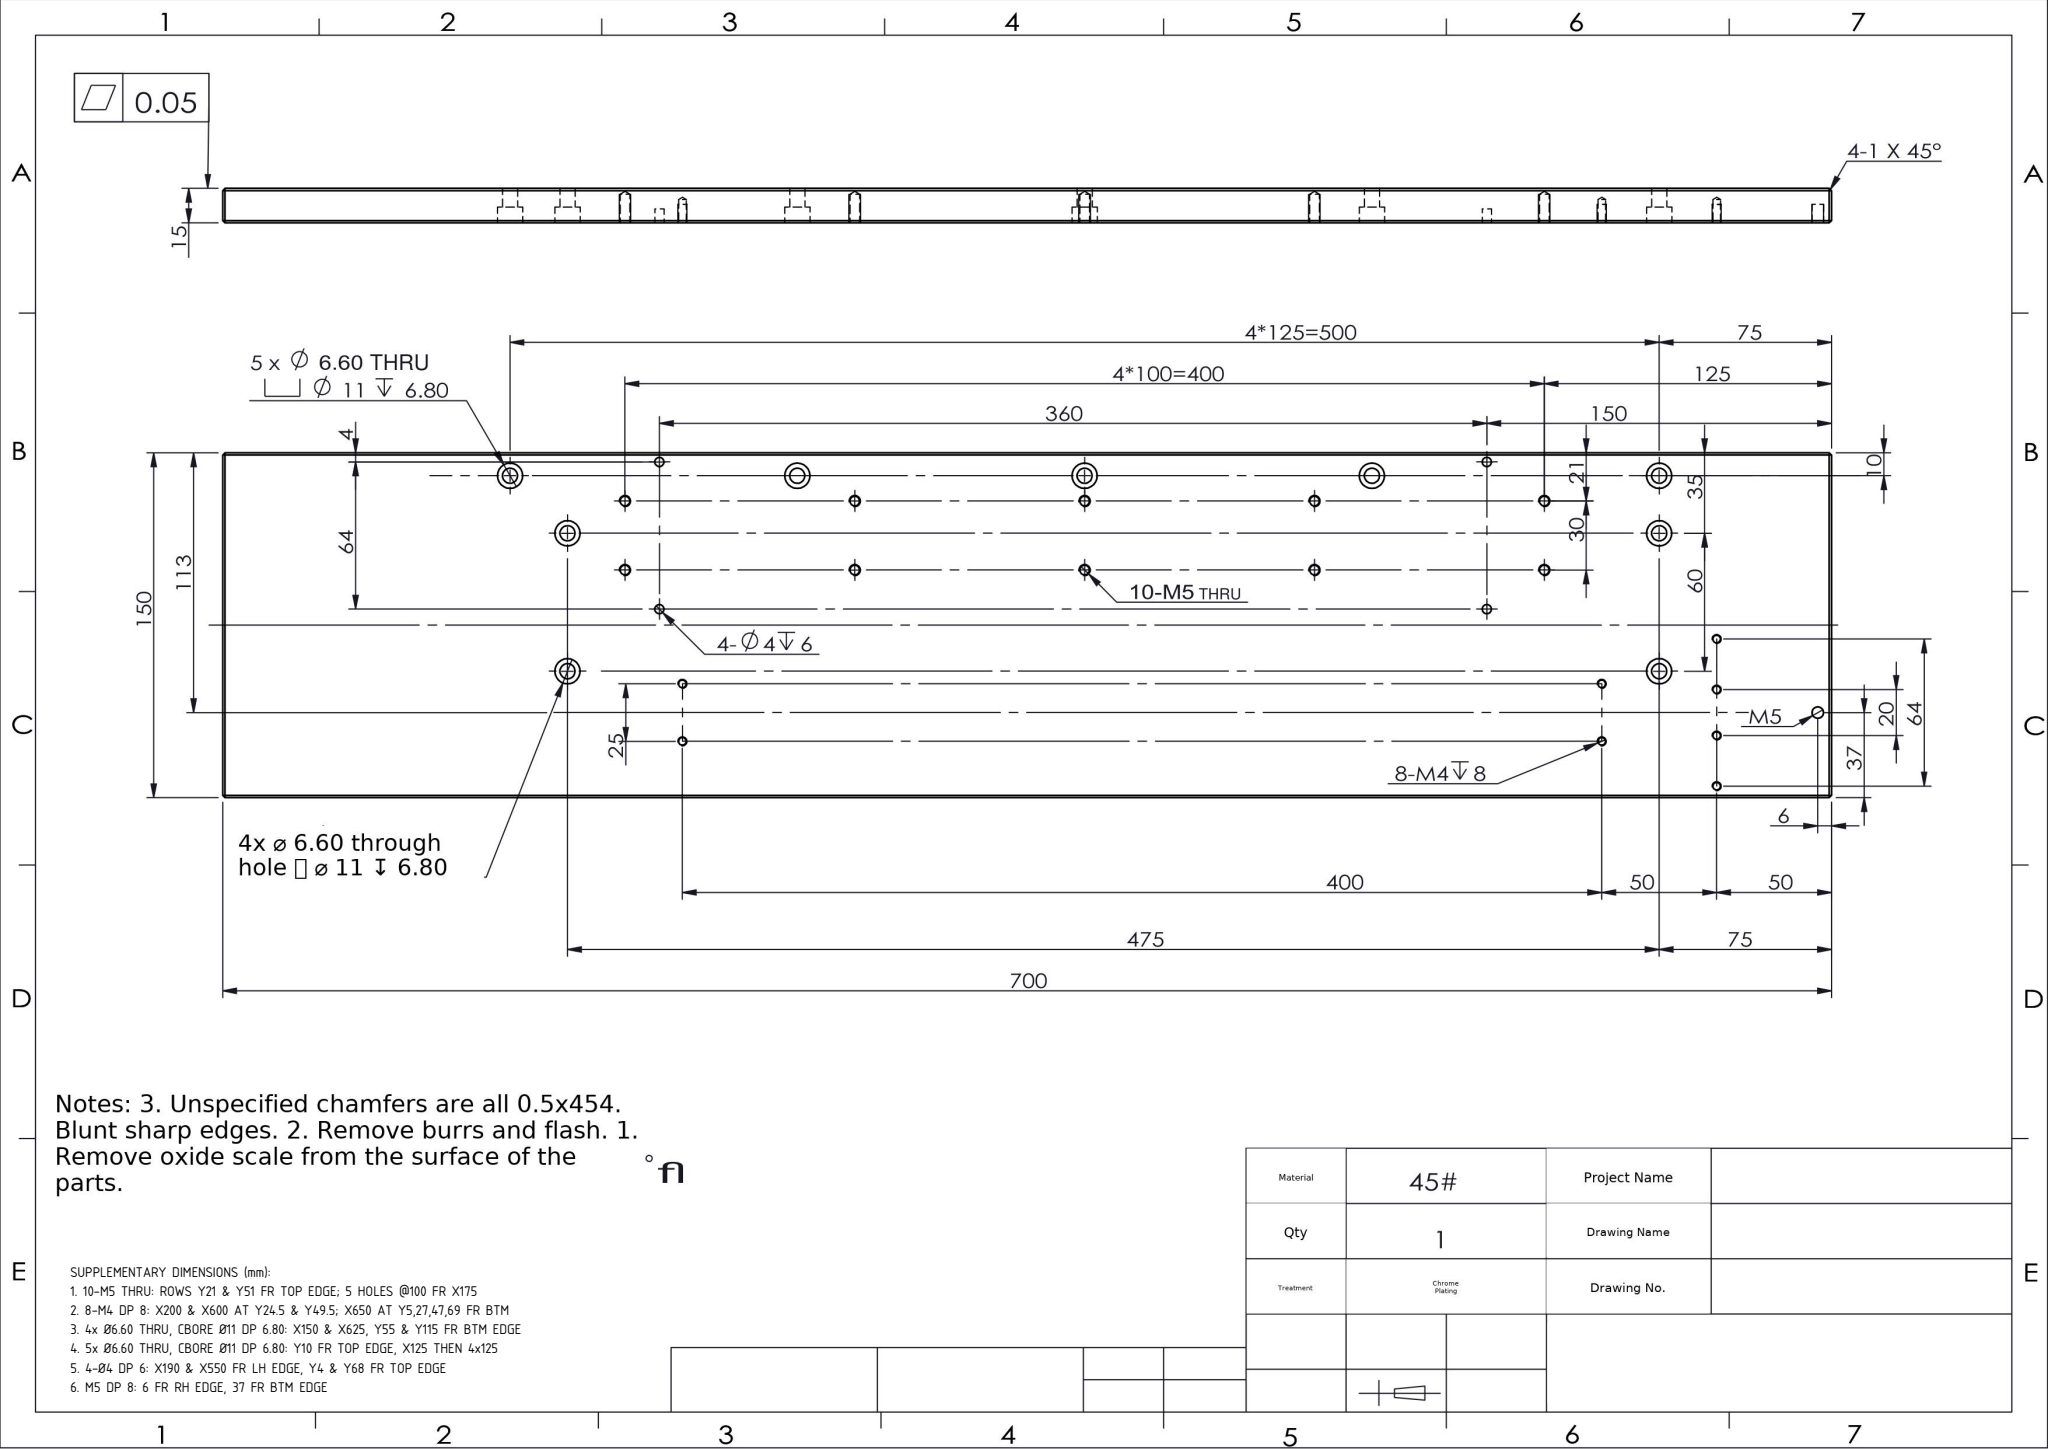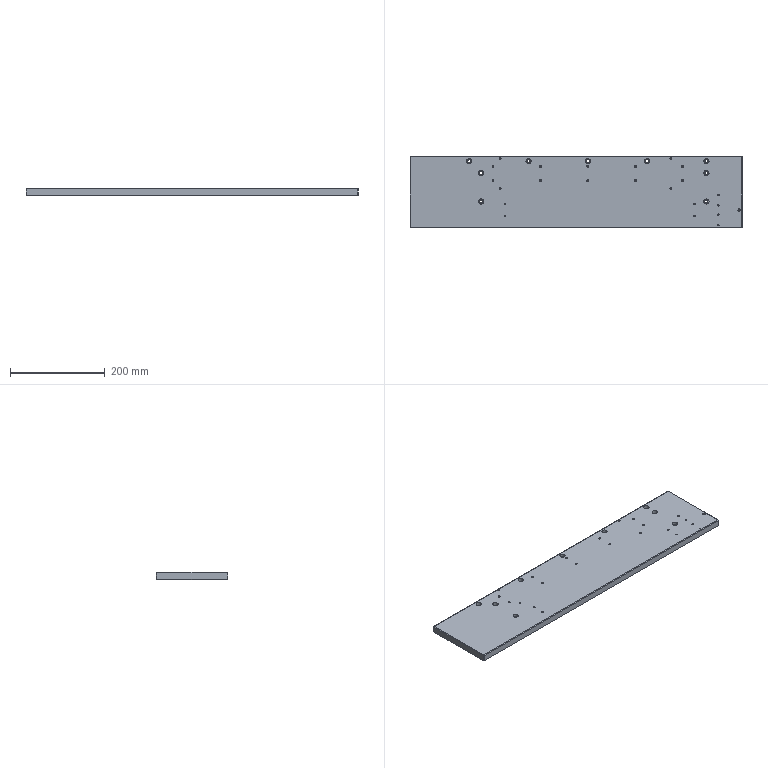Part | SolidWorks | mm | 1 solid | 158 faces | box 700 x 150 x 15 mm | volume 1561986 mm3 | cylinder 82 | plane 40 | cone 36 | commonest cylinder face diameters 4.2 x20 11 x18 6.6 x18 3.3 x16 4 x8 5 x2
build123d program:
from build123d import *

# Parameters (mm, degrees)
SKETCH1_W                                            = 700
SKETCH1_H                                            = 150
BOSS_EXTRUDE1_DEPTH                                  = 7.5
M5_TAPPED_HOLE1_AT_2_COUNT                           = 2
M5_TAPPED_HOLE1_AT_2_PITCH                           = 30
LPATTERN1_COUNT                                      = 5
LPATTERN1_PITCH                                      = 100
CHAMFER1_SIZE                                        = 1
HOLE_SIZE_ACCORDING_TO_THE_TYPE_OF_HEXAG_D           = 6.6
HOLE_SIZE_ACCORDING_TO_THE_TYPE_OF_HEXAG_CBORE_D     = 11
HOLE_SIZE_ACCORDING_TO_THE_TYPE_OF_HEXAG_CBORE_DEPTH = 6.8
SKETCH7_R                                            = 2
CUT_EXTRUDE1_DEPTH                                   = 6
M4_TAPPED_HOLE1_D                                    = 3.3
M4_TAPPED_HOLE1_DEPTH                                = 10.1
M4_TAPPED_HOLE1_TIP                                  = 0.9914
M4_TAPPED_HOLE2_AT_2_COUNT                           = 2
M4_TAPPED_HOLE2_AT_2_PITCH                           = 25
LPATTERN3_COUNT                                      = 2
LPATTERN3_PITCH                                      = 400
M4_TAPPED_HOLE4_D                                    = 3.3
M4_TAPPED_HOLE4_DEPTH                                = 10.1
M4_TAPPED_HOLE4_TIP                                  = 0.9914
HOLE_SIZE_ACCORDING_TO_THE_TYPE_OF_H_2_D             = 6.6
HOLE_SIZE_ACCORDING_TO_THE_TYPE_OF_H_2_CBORE_D       = 11
HOLE_SIZE_ACCORDING_TO_THE_TYPE_OF_H_2_CBORE_DEPTH   = 6.8
SKETCH26_R                                           = 2.5
CUT_EXTRUDE7_DEPTH                                   = 8


with BuildPart() as part:
    # Sketch1 → Boss-Extrude1 (new, symmetric)
    with BuildSketch(Plane.XY):
        Rectangle(SKETCH1_W, SKETCH1_H)
    extrude(amount=BOSS_EXTRUDE1_DEPTH, both=True)

    # Sketch2 → M5 Tapped Hole1 (revolve, cut)
    with BuildSketch(Plane(origin=(-175, 54, 7.5), x_dir=(0, -1, 0), z_dir=(1, 0, 0))):
        Polygon((0, 0), (0, 13.662), (2.1, 12.4), (2.1, 0), align=None)
    m5_tapped_hole1 = revolve(axis=Axis((-175, 54, 13.85), (0, 0, -1)), mode=Mode.SUBTRACT)

    # M5 Tapped Hole1 at 2: M5 Tapped Hole1 ×2
    with Locations(*[(0, -i * M5_TAPPED_HOLE1_AT_2_PITCH, 0) for i in range(1, M5_TAPPED_HOLE1_AT_2_COUNT)]):
        add(m5_tapped_hole1, mode=Mode.SUBTRACT)

    # LPattern1: M5 Tapped Hole1 ×5
    with Locations(*[(i * LPATTERN1_PITCH, 0, 0) for i in range(1, LPATTERN1_COUNT)]):
        add(m5_tapped_hole1, mode=Mode.SUBTRACT)

    # LPattern1 copy 1 sketch → LPattern1 copy 1 (revolve, cut)
    with BuildSketch(Plane(origin=(-75, 24, 7.5), x_dir=(0, -1, 0), z_dir=(1, 0, 0))):
        Polygon((0, 0), (0, 13.662), (2.1, 12.4), (2.1, 0), align=None)
    revolve(axis=Axis((-75, 24, 13.85), (0, 0, -1)), mode=Mode.SUBTRACT)

    # LPattern1 copy 2 sketch → LPattern1 copy 2 (revolve, cut)
    with BuildSketch(Plane(origin=(25, 24, 7.5), x_dir=(0, -1, 0), z_dir=(1, 0, 0))):
        Polygon((0, 0), (0, 13.662), (2.1, 12.4), (2.1, 0), align=None)
    revolve(axis=Axis((25, 24, 13.85), (0, 0, -1)), mode=Mode.SUBTRACT)

    # LPattern1 copy 3 sketch → LPattern1 copy 3 (revolve, cut)
    with BuildSketch(Plane(origin=(125, 24, 7.5), x_dir=(0, -1, 0), z_dir=(1, 0, 0))):
        Polygon((0, 0), (0, 13.662), (2.1, 12.4), (2.1, 0), align=None)
    revolve(axis=Axis((125, 24, 13.85), (0, 0, -1)), mode=Mode.SUBTRACT)

    # LPattern1 copy 4 sketch → LPattern1 copy 4 (revolve, cut)
    with BuildSketch(Plane(origin=(225, 24, 7.5), x_dir=(0, -1, 0), z_dir=(1, 0, 0))):
        Polygon((0, 0), (0, 13.662), (2.1, 12.4), (2.1, 0), align=None)
    revolve(axis=Axis((225, 24, 13.85), (0, 0, -1)), mode=Mode.SUBTRACT)

    # Chamfer1
    chamfer1_edges = [part.edges().sort_by_distance(p)[0] for p in [
        (-350, 0, 7.5),
        (0, -75, 7.5),
        (350, 0, 7.5),
        (0, -75, -7.5),
        (-350, 0, -7.5),
        (0, 75, -7.5),
        (350, 0, -7.5),
        (0, 75, 7.5),
        (350, -75, 0),
        (-350, -75, 0),
        (-350, 75, 0),
        (350, 75, 0),
    ]]
    chamfer(chamfer1_edges, length=CHAMFER1_SIZE)

    # Hole Size according to the type of Hexag (through all)
    with Locations(Plane.XY.offset(7.5)):
        with Locations((-225, 65), (275, 65), (25, 65), (-100, 65), (150, 65)):
            CounterBoreHole(HOLE_SIZE_ACCORDING_TO_THE_TYPE_OF_HEXAG_D / 2, HOLE_SIZE_ACCORDING_TO_THE_TYPE_OF_HEXAG_CBORE_D / 2, HOLE_SIZE_ACCORDING_TO_THE_TYPE_OF_HEXAG_CBORE_DEPTH)

    # Sketch7 → Cut-Extrude1 (cut)
    with BuildSketch(Plane.XY.offset(7.5)):
        with Locations((-160, 71)):
            Circle(SKETCH7_R)
        with Locations(Location((200, 71, 0), (0, 0, 180))):
            Circle(SKETCH7_R)
        with Locations((200, 7)):
            Circle(SKETCH7_R)
        with Locations((-160, 7)):
            Circle(SKETCH7_R)
    extrude(amount=-CUT_EXTRUDE1_DEPTH, mode=Mode.SUBTRACT)

    # M4 Tapped Hole1
    with Locations(Plane.XY.offset(7.5)):
        with Locations((300, -6), (300, -70)):
            Hole(M4_TAPPED_HOLE1_D / 2, depth=M4_TAPPED_HOLE1_DEPTH)
            with Locations((0, 0, -(M4_TAPPED_HOLE1_DEPTH + M4_TAPPED_HOLE1_TIP / 2))):  # 118° drill point
                Cone(0, M4_TAPPED_HOLE1_D / 2, M4_TAPPED_HOLE1_TIP, mode=Mode.SUBTRACT)

    # Sketch17 → M4 Tapped Hole2 (revolve, cut)
    with BuildSketch(Plane(origin=(250, -25.5, 7.5), x_dir=(0, -1, 0), z_dir=(1, 0, 0))):
        Polygon((0, 0), (0, 11.091), (1.65, 10.1), (1.65, 0), align=None)
    m4_tapped_hole2 = revolve(axis=Axis((250, -25.5, 13.85), (0, 0, -1)), mode=Mode.SUBTRACT)

    # M4 Tapped Hole2 at 2: M4 Tapped Hole2 ×2
    with Locations(*[(0, -i * M4_TAPPED_HOLE2_AT_2_PITCH, 0) for i in range(1, M4_TAPPED_HOLE2_AT_2_COUNT)]):
        add(m4_tapped_hole2, mode=Mode.SUBTRACT)

    # LPattern3: M4 Tapped Hole2 ×2
    with Locations(*[(-i * LPATTERN3_PITCH, 0, 0) for i in range(1, LPATTERN3_COUNT)]):
        add(m4_tapped_hole2, mode=Mode.SUBTRACT)

    # LPattern3 copy 1 sketch → LPattern3 copy 1 (revolve, cut)
    with BuildSketch(Plane(origin=(-150, -50.5, 7.5), x_dir=(0, -1, 0), z_dir=(1, 0, 0))):
        Polygon((0, 0), (0, 11.091), (1.65, 10.1), (1.65, 0), align=None)
    revolve(axis=Axis((-150, -50.5, 13.85), (0, 0, -1)), mode=Mode.SUBTRACT)

    # M4 Tapped Hole4
    with Locations(Plane.XY.offset(7.5)):
        with Locations((300, -28), (300, -48)):
            Hole(M4_TAPPED_HOLE4_D / 2, depth=M4_TAPPED_HOLE4_DEPTH)
            with Locations((0, 0, -(M4_TAPPED_HOLE4_DEPTH + M4_TAPPED_HOLE4_TIP / 2))):  # 118° drill point
                Cone(0, M4_TAPPED_HOLE4_D / 2, M4_TAPPED_HOLE4_TIP, mode=Mode.SUBTRACT)

    # Hole Size according to the type of H 2 (through all)
    with Locations(Plane.XY.offset(7.5)):
        with Locations((-200, 40), (-200, -20), (275, 40), (275, -20)):
            CounterBoreHole(HOLE_SIZE_ACCORDING_TO_THE_TYPE_OF_H_2_D / 2, HOLE_SIZE_ACCORDING_TO_THE_TYPE_OF_H_2_CBORE_D / 2, HOLE_SIZE_ACCORDING_TO_THE_TYPE_OF_H_2_CBORE_DEPTH)

    # Sketch26 → Cut-Extrude7 (cut)
    with BuildSketch(Plane.XY.offset(7.5)):
        with Locations((344, -38)):
            Circle(SKETCH26_R)
    extrude(amount=-CUT_EXTRUDE7_DEPTH, mode=Mode.SUBTRACT)


solid = part.part